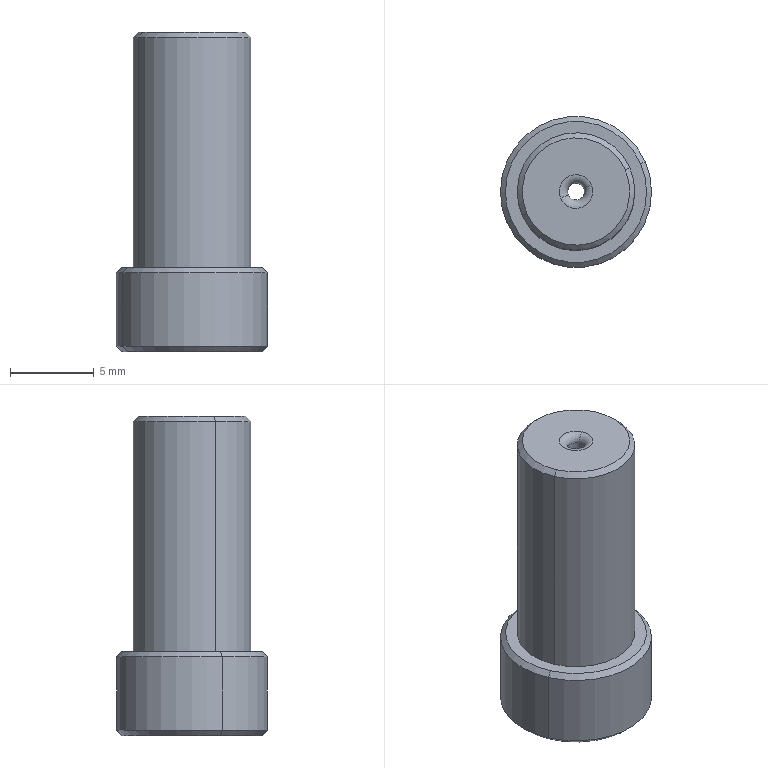Component | SolidWorks | AS-011-JG0135-1 | 1 solid | 19 faces | box 9 x 9 x 19 mm | volume 824 mm3 | cylinder 6 | cone 6 | torus 4 | plane 3 | commonest cylinder face diameters 1 x2 7 x2 9 x2
build123d program:
from build123d import *


with BuildPart() as part:
    # Sketch1 → Revolve1 (revolve)
    with BuildSketch(Plane.XY, mode=Mode.PRIVATE) as revolve1_sk:
        with BuildLine():
            Line((-4.938, 0.5), (-20.438, 0.5))
            ThreePointArc((-20.438, 0.5), (-20.792, 0.6464), (-20.938, 1))
            Line((-20.938, 1), (-20.938, 3.2))
            Line((-20.938, 3.2), (-20.638, 3.5))
            Line((-20.638, 3.5), (-6.938, 3.5))
            Line((-6.938, 3.5), (-6.938, 4.2))
            Line((-6.938, 4.2), (-6.638, 4.5))
            Line((-6.638, 4.5), (-2.238, 4.5))
            Line((-2.238, 4.5), (-1.938, 4.2))
            Line((-1.938, 4.2), (-1.938, 3.5))
            ThreePointArc((-1.938, 3.5), (-2.817, 1.379), (-4.938, 0.5))
        make_face()
    revolve(revolve1_sk.sketch.rotate(Axis((-20.938, 0, 0), (1, 0, 0)), 90), axis=Axis((-20.938, 0, 0), (1, 0, 0)))


solid = part.part

# Placed as in the assembly
solid = solid.moved(Location((-15, -28, -44.438), (0, 90, 0)))
STEP:
#1=COLOUR_RGB('',0.7922,0.8196,0.9333);
#2=FILL_AREA_STYLE_COLOUR('',#1);
#3=FILL_AREA_STYLE('',(#2));
#4=SURFACE_STYLE_FILL_AREA(#3);
#5=SURFACE_SIDE_STYLE('',(#4));
#6=SURFACE_STYLE_USAGE(.BOTH.,#5);
#7=PRESENTATION_STYLE_ASSIGNMENT((#6));
#8=CARTESIAN_POINT('',(-0.6086,-1.11,-1.555));
#9=VERTEX_POINT('',#8);
#10=CARTESIAN_POINT('',(-0.5725,-1.094,-1.555));
#11=VERTEX_POINT('',#10);
#12=CARTESIAN_POINT('',(-0.5906,-1.102,-1.555));
#13=DIRECTION('',(0.,0.,1.));
#14=DIRECTION('',(0.9157,0.4019,0.));
#15=AXIS2_PLACEMENT_3D('',#12,#13,#14);
#16=CIRCLE('',#15,0.01969);
#17=EDGE_CURVE('',#9,#11,#16,.T.);
#18=ORIENTED_EDGE('',*,*,#17,.F.);
#19=CARTESIAN_POINT('',(-0.6086,-1.11,-0.9449));
#20=VERTEX_POINT('',#19);
#21=CARTESIAN_POINT('',(-0.6086,-1.11,-0.9252));
#22=DIRECTION('',(0.,0.,1.));
#23=VECTOR('',#22,39.37);
#24=LINE('',#21,#23);
#25=EDGE_CURVE('',#9,#20,#24,.T.);
#26=ORIENTED_EDGE('',*,*,#25,.T.);
#27=CARTESIAN_POINT('',(-0.5725,-1.094,-0.9449));
#28=VERTEX_POINT('',#27);
#29=CARTESIAN_POINT('',(-0.5906,-1.102,-0.9449));
#30=DIRECTION('',(0.,0.,1.));
#31=DIRECTION('',(0.9157,0.4019,0.));
#32=AXIS2_PLACEMENT_3D('',#29,#30,#31);
#33=CIRCLE('',#32,0.01969);
#34=EDGE_CURVE('',#20,#28,#33,.T.);
#35=ORIENTED_EDGE('',*,*,#34,.T.);
#36=CARTESIAN_POINT('',(-0.5725,-1.094,-0.9252));
#37=DIRECTION('',(0.,0.,1.));
#38=VECTOR('',#37,39.37);
#39=LINE('',#36,#38);
#40=EDGE_CURVE('',#11,#28,#39,.T.);
#41=ORIENTED_EDGE('',*,*,#40,.F.);
#42=EDGE_LOOP('',(#18,#26,#35,#41));
#43=FACE_OUTER_BOUND('',#42,.T.);
#44=CARTESIAN_POINT('',(-0.5906,-1.102,-0.9252));
#45=DIRECTION('',(0.,0.,1.));
#46=DIRECTION('',(0.9157,0.4019,0.));
#47=AXIS2_PLACEMENT_3D('',#44,#45,#46);
#48=CYLINDRICAL_SURFACE('',#47,0.01969);
#49=ADVANCED_FACE('',(#43),#48,.F.);
#50=CARTESIAN_POINT('',(-0.5545,-1.087,-0.9252));
#51=VERTEX_POINT('',#50);
#52=CARTESIAN_POINT('',(-0.6266,-1.118,-0.9252));
#53=VERTEX_POINT('',#52);
#54=CARTESIAN_POINT('',(-0.5906,-1.102,-0.9252));
#55=DIRECTION('',(0.,0.,1.));
#56=DIRECTION('',(0.9157,0.4019,0.));
#57=AXIS2_PLACEMENT_3D('',#54,#55,#56);
#58=CIRCLE('',#57,0.03937);
#59=EDGE_CURVE('',#51,#53,#58,.T.);
#60=ORIENTED_EDGE('',*,*,#59,.T.);
#61=CARTESIAN_POINT('',(-0.6266,-1.118,-0.9449));
#62=DIRECTION('',(-0.4019,0.9157,-0.));
#63=DIRECTION('',(-0.9157,-0.4019,0.));
#64=AXIS2_PLACEMENT_3D('',#61,#62,#63);
#65=CIRCLE('',#64,0.01969);
#66=EDGE_CURVE('',#53,#20,#65,.T.);
#67=ORIENTED_EDGE('',*,*,#66,.T.);
#68=CARTESIAN_POINT('',(-0.5906,-1.102,-0.9449));
#69=DIRECTION('',(0.,0.,1.));
#70=DIRECTION('',(0.9157,0.4019,0.));
#71=AXIS2_PLACEMENT_3D('',#68,#69,#70);
#72=CIRCLE('',#71,0.01969);
#73=EDGE_CURVE('',#28,#20,#72,.T.);
#74=ORIENTED_EDGE('',*,*,#73,.F.);
#75=CARTESIAN_POINT('',(-0.5545,-1.087,-0.9449));
#76=DIRECTION('',(0.4019,-0.9157,0.));
#77=DIRECTION('',(0.9157,0.4019,0.));
#78=AXIS2_PLACEMENT_3D('',#75,#76,#77);
#79=CIRCLE('',#78,0.01969);
#80=EDGE_CURVE('',#51,#28,#79,.T.);
#81=ORIENTED_EDGE('',*,*,#80,.F.);
#82=EDGE_LOOP('',(#60,#67,#74,#81));
#83=FACE_OUTER_BOUND('',#82,.T.);
#84=CARTESIAN_POINT('',(-0.5906,-1.102,-0.9449));
#85=DIRECTION('',(0.,0.,1.));
#86=DIRECTION('',(0.9157,0.4019,-0.));
#87=AXIS2_PLACEMENT_3D('',#84,#85,#86);
#88=TOROIDAL_SURFACE('',#87,0.03937,0.01969);
#89=ADVANCED_FACE('',(#83),#88,.T.);
#90=CARTESIAN_POINT('',(-0.4752,-1.052,-0.9252));
#91=VERTEX_POINT('',#90);
#92=CARTESIAN_POINT('',(-0.7059,-1.153,-0.9252));
#93=VERTEX_POINT('',#92);
#94=CARTESIAN_POINT('',(-0.5906,-1.102,-0.9252));
#95=DIRECTION('',(0.,0.,1.));
#96=DIRECTION('',(0.9157,0.4019,0.));
#97=AXIS2_PLACEMENT_3D('',#94,#95,#96);
#98=CIRCLE('',#97,0.126);
#99=EDGE_CURVE('',#91,#93,#98,.T.);
#100=ORIENTED_EDGE('',*,*,#99,.F.);
#101=CARTESIAN_POINT('',(-0.4644,-1.047,-0.937));
#102=VERTEX_POINT('',#101);
#103=CARTESIAN_POINT('',(-0.4644,-1.047,-0.937));
#104=DIRECTION('',(0.6475,0.2842,-0.7071));
#105=VECTOR('',#104,39.37);
#106=LINE('',#103,#105);
#107=EDGE_CURVE('',#91,#102,#106,.T.);
#108=ORIENTED_EDGE('',*,*,#107,.T.);
#109=CARTESIAN_POINT('',(-0.7167,-1.158,-0.937));
#110=VERTEX_POINT('',#109);
#111=CARTESIAN_POINT('',(-0.5906,-1.102,-0.937));
#112=DIRECTION('',(0.,0.,1.));
#113=DIRECTION('',(0.9157,0.4019,0.));
#114=AXIS2_PLACEMENT_3D('',#111,#112,#113);
#115=CIRCLE('',#114,0.1378);
#116=EDGE_CURVE('',#102,#110,#115,.T.);
#117=ORIENTED_EDGE('',*,*,#116,.T.);
#118=CARTESIAN_POINT('',(-0.7167,-1.158,-0.937));
#119=DIRECTION('',(-0.6475,-0.2842,-0.7071));
#120=VECTOR('',#119,39.37);
#121=LINE('',#118,#120);
#122=EDGE_CURVE('',#93,#110,#121,.T.);
#123=ORIENTED_EDGE('',*,*,#122,.F.);
#124=EDGE_LOOP('',(#100,#108,#117,#123));
#125=FACE_OUTER_BOUND('',#124,.T.);
#126=CARTESIAN_POINT('',(-0.5906,-1.102,-0.937));
#127=DIRECTION('',(-0.,-0.,-1.));
#128=DIRECTION('',(-0.9157,-0.4019,0.));
#129=AXIS2_PLACEMENT_3D('',#126,#127,#128);
#130=CONICAL_SURFACE('',#129,0.1378,0.7854);
#131=ADVANCED_FACE('',(#125),#130,.T.);
#132=CARTESIAN_POINT('',(-0.4644,-1.047,-1.476));
#133=VERTEX_POINT('',#132);
#134=CARTESIAN_POINT('',(-0.7167,-1.158,-1.476));
#135=VERTEX_POINT('',#134);
#136=CARTESIAN_POINT('',(-0.5906,-1.102,-1.476));
#137=DIRECTION('',(0.,0.,1.));
#138=DIRECTION('',(0.9157,0.4019,0.));
#139=AXIS2_PLACEMENT_3D('',#136,#137,#138);
#140=CIRCLE('',#139,0.1378);
#141=EDGE_CURVE('',#133,#135,#140,.T.);
#142=ORIENTED_EDGE('',*,*,#141,.T.);
#143=CARTESIAN_POINT('',(-0.7167,-1.158,-0.9252));
#144=DIRECTION('',(0.,0.,1.));
#145=VECTOR('',#144,39.37);
#146=LINE('',#143,#145);
#147=EDGE_CURVE('',#135,#110,#146,.T.);
#148=ORIENTED_EDGE('',*,*,#147,.T.);
#149=ORIENTED_EDGE('',*,*,#116,.F.);
#150=CARTESIAN_POINT('',(-0.4644,-1.047,-0.9252));
#151=DIRECTION('',(0.,0.,1.));
#152=VECTOR('',#151,39.37);
#153=LINE('',#150,#152);
#154=EDGE_CURVE('',#133,#102,#153,.T.);
#155=ORIENTED_EDGE('',*,*,#154,.F.);
#156=EDGE_LOOP('',(#142,#148,#149,#155));
#157=FACE_OUTER_BOUND('',#156,.T.);
#158=CARTESIAN_POINT('',(-0.5906,-1.102,-0.9252));
#159=DIRECTION('',(0.,0.,1.));
#160=DIRECTION('',(0.9157,0.4019,0.));
#161=AXIS2_PLACEMENT_3D('',#158,#159,#160);
#162=CYLINDRICAL_SURFACE('',#161,0.1378);
#163=ADVANCED_FACE('',(#157),#162,.T.);
#164=CARTESIAN_POINT('',(-0.4391,-1.036,-1.476));
#165=VERTEX_POINT('',#164);
#166=CARTESIAN_POINT('',(-0.742,-1.169,-1.476));
#167=VERTEX_POINT('',#166);
#168=CARTESIAN_POINT('',(-0.5906,-1.102,-1.476));
#169=DIRECTION('',(0.,0.,1.));
#170=DIRECTION('',(0.9157,0.4019,0.));
#171=AXIS2_PLACEMENT_3D('',#168,#169,#170);
#172=CIRCLE('',#171,0.1654);
#173=EDGE_CURVE('',#165,#167,#172,.T.);
#174=ORIENTED_EDGE('',*,*,#173,.F.);
#175=CARTESIAN_POINT('',(-0.4283,-1.031,-1.488));
#176=VERTEX_POINT('',#175);
#177=CARTESIAN_POINT('',(-0.4283,-1.031,-1.488));
#178=DIRECTION('',(0.6475,0.2842,-0.7071));
#179=VECTOR('',#178,39.37);
#180=LINE('',#177,#179);
#181=EDGE_CURVE('',#165,#176,#180,.T.);
#182=ORIENTED_EDGE('',*,*,#181,.T.);
#183=CARTESIAN_POINT('',(-0.7528,-1.174,-1.488));
#184=VERTEX_POINT('',#183);
#185=CARTESIAN_POINT('',(-0.5906,-1.102,-1.488));
#186=DIRECTION('',(0.,0.,1.));
#187=DIRECTION('',(0.9157,0.4019,0.));
#188=AXIS2_PLACEMENT_3D('',#185,#186,#187);
#189=CIRCLE('',#188,0.1772);
#190=EDGE_CURVE('',#176,#184,#189,.T.);
#191=ORIENTED_EDGE('',*,*,#190,.T.);
#192=CARTESIAN_POINT('',(-0.7528,-1.174,-1.488));
#193=DIRECTION('',(-0.6475,-0.2842,-0.7071));
#194=VECTOR('',#193,39.37);
#195=LINE('',#192,#194);
#196=EDGE_CURVE('',#167,#184,#195,.T.);
#197=ORIENTED_EDGE('',*,*,#196,.F.);
#198=EDGE_LOOP('',(#174,#182,#191,#197));
#199=FACE_OUTER_BOUND('',#198,.T.);
#200=CARTESIAN_POINT('',(-0.5906,-1.102,-1.488));
#201=DIRECTION('',(-0.,-0.,-1.));
#202=DIRECTION('',(-0.9157,-0.4019,0.));
#203=AXIS2_PLACEMENT_3D('',#200,#201,#202);
#204=CONICAL_SURFACE('',#203,0.1772,0.7854);
#205=ADVANCED_FACE('',(#199),#204,.T.);
#206=CARTESIAN_POINT('',(-0.4283,-1.031,-1.661));
#207=VERTEX_POINT('',#206);
#208=CARTESIAN_POINT('',(-0.7528,-1.174,-1.661));
#209=VERTEX_POINT('',#208);
#210=CARTESIAN_POINT('',(-0.5906,-1.102,-1.661));
#211=DIRECTION('',(0.,0.,1.));
#212=DIRECTION('',(0.9157,0.4019,0.));
#213=AXIS2_PLACEMENT_3D('',#210,#211,#212);
#214=CIRCLE('',#213,0.1772);
#215=EDGE_CURVE('',#207,#209,#214,.T.);
#216=ORIENTED_EDGE('',*,*,#215,.T.);
#217=CARTESIAN_POINT('',(-0.7528,-1.174,-0.9252));
#218=DIRECTION('',(0.,0.,1.));
#219=VECTOR('',#218,39.37);
#220=LINE('',#217,#219);
#221=EDGE_CURVE('',#209,#184,#220,.T.);
#222=ORIENTED_EDGE('',*,*,#221,.T.);
#223=ORIENTED_EDGE('',*,*,#190,.F.);
#224=CARTESIAN_POINT('',(-0.4283,-1.031,-0.9252));
#225=DIRECTION('',(0.,0.,1.));
#226=VECTOR('',#225,39.37);
#227=LINE('',#224,#226);
#228=EDGE_CURVE('',#207,#176,#227,.T.);
#229=ORIENTED_EDGE('',*,*,#228,.F.);
#230=EDGE_LOOP('',(#216,#222,#223,#229));
#231=FACE_OUTER_BOUND('',#230,.T.);
#232=CARTESIAN_POINT('',(-0.5906,-1.102,-0.9252));
#233=DIRECTION('',(0.,0.,1.));
#234=DIRECTION('',(0.9157,0.4019,0.));
#235=AXIS2_PLACEMENT_3D('',#232,#233,#234);
#236=CYLINDRICAL_SURFACE('',#235,0.1772);
#237=ADVANCED_FACE('',(#231),#236,.T.);
#238=CARTESIAN_POINT('',(-0.4391,-1.036,-1.673));
#239=VERTEX_POINT('',#238);
#240=CARTESIAN_POINT('',(-0.742,-1.169,-1.673));
#241=VERTEX_POINT('',#240);
#242=CARTESIAN_POINT('',(-0.5906,-1.102,-1.673));
#243=DIRECTION('',(0.,0.,1.));
#244=DIRECTION('',(0.9157,0.4019,0.));
#245=AXIS2_PLACEMENT_3D('',#242,#243,#244);
#246=CIRCLE('',#245,0.1654);
#247=EDGE_CURVE('',#239,#241,#246,.T.);
#248=ORIENTED_EDGE('',*,*,#247,.T.);
#249=CARTESIAN_POINT('',(-0.742,-1.169,-1.673));
#250=DIRECTION('',(-0.6475,-0.2842,0.7071));
#251=VECTOR('',#250,39.37);
#252=LINE('',#249,#251);
#253=EDGE_CURVE('',#241,#209,#252,.T.);
#254=ORIENTED_EDGE('',*,*,#253,.T.);
#255=ORIENTED_EDGE('',*,*,#215,.F.);
#256=CARTESIAN_POINT('',(-0.4391,-1.036,-1.673));
#257=DIRECTION('',(0.6475,0.2842,0.7071));
#258=VECTOR('',#257,39.37);
#259=LINE('',#256,#258);
#260=EDGE_CURVE('',#239,#207,#259,.T.);
#261=ORIENTED_EDGE('',*,*,#260,.F.);
#262=EDGE_LOOP('',(#248,#254,#255,#261));
#263=FACE_OUTER_BOUND('',#262,.T.);
#264=CARTESIAN_POINT('',(-0.5906,-1.102,-1.673));
#265=DIRECTION('',(0.,0.,1.));
#266=DIRECTION('',(0.9157,0.4019,0.));
#267=AXIS2_PLACEMENT_3D('',#264,#265,#266);
#268=CONICAL_SURFACE('',#267,0.1654,0.7854);
#269=ADVANCED_FACE('',(#263),#268,.T.);
#270=CARTESIAN_POINT('',(-0.5906,-1.102,-1.555));
#271=DIRECTION('',(0.,0.,1.));
#272=DIRECTION('',(0.9157,0.4019,0.));
#273=AXIS2_PLACEMENT_3D('',#270,#271,#272);
#274=CIRCLE('',#273,0.01969);
#275=EDGE_CURVE('',#11,#9,#274,.T.);
#276=ORIENTED_EDGE('',*,*,#275,.T.);
#277=CARTESIAN_POINT('',(-0.7167,-1.158,-1.673));
#278=VERTEX_POINT('',#277);
#279=CARTESIAN_POINT('',(-0.7167,-1.158,-1.555));
#280=DIRECTION('',(-0.4019,0.9157,-0.));
#281=DIRECTION('',(-0.9157,-0.4019,0.));
#282=AXIS2_PLACEMENT_3D('',#279,#280,#281);
#283=CIRCLE('',#282,0.1181);
#284=EDGE_CURVE('',#9,#278,#283,.T.);
#285=ORIENTED_EDGE('',*,*,#284,.T.);
#286=CARTESIAN_POINT('',(-0.4644,-1.047,-1.673));
#287=VERTEX_POINT('',#286);
#288=CARTESIAN_POINT('',(-0.5906,-1.102,-1.673));
#289=DIRECTION('',(0.,0.,1.));
#290=DIRECTION('',(0.9157,0.4019,0.));
#291=AXIS2_PLACEMENT_3D('',#288,#289,#290);
#292=CIRCLE('',#291,0.1378);
#293=EDGE_CURVE('',#287,#278,#292,.T.);
#294=ORIENTED_EDGE('',*,*,#293,.F.);
#295=CARTESIAN_POINT('',(-0.4644,-1.047,-1.555));
#296=DIRECTION('',(0.4019,-0.9157,0.));
#297=DIRECTION('',(0.9157,0.4019,0.));
#298=AXIS2_PLACEMENT_3D('',#295,#296,#297);
#299=CIRCLE('',#298,0.1181);
#300=EDGE_CURVE('',#11,#287,#299,.T.);
#301=ORIENTED_EDGE('',*,*,#300,.F.);
#302=EDGE_LOOP('',(#276,#285,#294,#301));
#303=FACE_OUTER_BOUND('',#302,.T.);
#304=CARTESIAN_POINT('',(-0.5906,-1.102,-1.555));
#305=DIRECTION('',(0.,0.,1.));
#306=DIRECTION('',(0.9157,0.4019,-0.));
#307=AXIS2_PLACEMENT_3D('',#304,#305,#306);
#308=TOROIDAL_SURFACE('',#307,0.1378,0.1181);
#309=ADVANCED_FACE('',(#303),#308,.T.);
#310=ORIENTED_EDGE('',*,*,#284,.F.);
#311=ORIENTED_EDGE('',*,*,#17,.T.);
#312=ORIENTED_EDGE('',*,*,#300,.T.);
#313=CARTESIAN_POINT('',(-0.5906,-1.102,-1.673));
#314=DIRECTION('',(0.,0.,1.));
#315=DIRECTION('',(0.9157,0.4019,0.));
#316=AXIS2_PLACEMENT_3D('',#313,#314,#315);
#317=CIRCLE('',#316,0.1378);
#318=EDGE_CURVE('',#278,#287,#317,.T.);
#319=ORIENTED_EDGE('',*,*,#318,.F.);
#320=EDGE_LOOP('',(#310,#311,#312,#319));
#321=FACE_OUTER_BOUND('',#320,.T.);
#322=CARTESIAN_POINT('',(-0.5906,-1.102,-1.555));
#323=DIRECTION('',(0.,0.,1.));
#324=DIRECTION('',(0.9157,0.4019,-0.));
#325=AXIS2_PLACEMENT_3D('',#322,#323,#324);
#326=TOROIDAL_SURFACE('',#325,0.1378,0.1181);
#327=ADVANCED_FACE('',(#321),#326,.T.);
#328=ORIENTED_EDGE('',*,*,#247,.F.);
#329=CARTESIAN_POINT('',(-0.5906,-1.102,-1.673));
#330=DIRECTION('',(0.,0.,1.));
#331=DIRECTION('',(0.9157,0.4019,0.));
#332=AXIS2_PLACEMENT_3D('',#329,#330,#331);
#333=CIRCLE('',#332,0.1654);
#334=EDGE_CURVE('',#241,#239,#333,.T.);
#335=ORIENTED_EDGE('',*,*,#334,.F.);
#336=EDGE_LOOP('',(#328,#335));
#337=FACE_OUTER_BOUND('',#336,.T.);
#338=ORIENTED_EDGE('',*,*,#293,.T.);
#339=ORIENTED_EDGE('',*,*,#318,.T.);
#340=EDGE_LOOP('',(#338,#339));
#341=FACE_BOUND('',#340,.T.);
#342=CARTESIAN_POINT('',(-0.657,-0.951,-1.673));
#343=DIRECTION('',(-0.,0.,1.));
#344=DIRECTION('',(0.9157,0.4019,-0.));
#345=AXIS2_PLACEMENT_3D('',#342,#343,#344);
#346=PLANE('',#345);
#347=ADVANCED_FACE('',(#337,#341),#346,.F.);
#348=ORIENTED_EDGE('',*,*,#253,.F.);
#349=ORIENTED_EDGE('',*,*,#334,.T.);
#350=ORIENTED_EDGE('',*,*,#260,.T.);
#351=CARTESIAN_POINT('',(-0.5906,-1.102,-1.661));
#352=DIRECTION('',(0.,0.,1.));
#353=DIRECTION('',(0.9157,0.4019,0.));
#354=AXIS2_PLACEMENT_3D('',#351,#352,#353);
#355=CIRCLE('',#354,0.1772);
#356=EDGE_CURVE('',#209,#207,#355,.T.);
#357=ORIENTED_EDGE('',*,*,#356,.F.);
#358=EDGE_LOOP('',(#348,#349,#350,#357));
#359=FACE_OUTER_BOUND('',#358,.T.);
#360=CARTESIAN_POINT('',(-0.5906,-1.102,-1.673));
#361=DIRECTION('',(0.,0.,1.));
#362=DIRECTION('',(0.9157,0.4019,0.));
#363=AXIS2_PLACEMENT_3D('',#360,#361,#362);
#364=CONICAL_SURFACE('',#363,0.1654,0.7854);
#365=ADVANCED_FACE('',(#359),#364,.T.);
#366=ORIENTED_EDGE('',*,*,#221,.F.);
#367=ORIENTED_EDGE('',*,*,#356,.T.);
#368=ORIENTED_EDGE('',*,*,#228,.T.);
#369=CARTESIAN_POINT('',(-0.5906,-1.102,-1.488));
#370=DIRECTION('',(0.,0.,1.));
#371=DIRECTION('',(0.9157,0.4019,0.));
#372=AXIS2_PLACEMENT_3D('',#369,#370,#371);
#373=CIRCLE('',#372,0.1772);
#374=EDGE_CURVE('',#184,#176,#373,.T.);
#375=ORIENTED_EDGE('',*,*,#374,.F.);
#376=EDGE_LOOP('',(#366,#367,#368,#375));
#377=FACE_OUTER_BOUND('',#376,.T.);
#378=CARTESIAN_POINT('',(-0.5906,-1.102,-0.9252));
#379=DIRECTION('',(0.,0.,1.));
#380=DIRECTION('',(0.9157,0.4019,0.));
#381=AXIS2_PLACEMENT_3D('',#378,#379,#380);
#382=CYLINDRICAL_SURFACE('',#381,0.1772);
#383=ADVANCED_FACE('',(#377),#382,.T.);
#384=ORIENTED_EDGE('',*,*,#181,.F.);
#385=CARTESIAN_POINT('',(-0.5906,-1.102,-1.476));
#386=DIRECTION('',(0.,0.,1.));
#387=DIRECTION('',(0.9157,0.4019,0.));
#388=AXIS2_PLACEMENT_3D('',#385,#386,#387);
#389=CIRCLE('',#388,0.1654);
#390=EDGE_CURVE('',#167,#165,#389,.T.);
#391=ORIENTED_EDGE('',*,*,#390,.F.);
#392=ORIENTED_EDGE('',*,*,#196,.T.);
#393=ORIENTED_EDGE('',*,*,#374,.T.);
#394=EDGE_LOOP('',(#384,#391,#392,#393));
#395=FACE_OUTER_BOUND('',#394,.T.);
#396=CARTESIAN_POINT('',(-0.5906,-1.102,-1.488));
#397=DIRECTION('',(-0.,-0.,-1.));
#398=DIRECTION('',(-0.9157,-0.4019,0.));
#399=AXIS2_PLACEMENT_3D('',#396,#397,#398);
#400=CONICAL_SURFACE('',#399,0.1772,0.7854);
#401=ADVANCED_FACE('',(#395),#400,.T.);
#402=ORIENTED_EDGE('',*,*,#141,.F.);
#403=CARTESIAN_POINT('',(-0.5906,-1.102,-1.476));
#404=DIRECTION('',(0.,0.,1.));
#405=DIRECTION('',(0.9157,0.4019,0.));
#406=AXIS2_PLACEMENT_3D('',#403,#404,#405);
#407=CIRCLE('',#406,0.1378);
#408=EDGE_CURVE('',#135,#133,#407,.T.);
#409=ORIENTED_EDGE('',*,*,#408,.F.);
#410=EDGE_LOOP('',(#402,#409));
#411=FACE_BOUND('',#410,.T.);
#412=ORIENTED_EDGE('',*,*,#390,.T.);
#413=ORIENTED_EDGE('',*,*,#173,.T.);
#414=EDGE_LOOP('',(#412,#413));
#415=FACE_OUTER_BOUND('',#414,.T.);
#416=CARTESIAN_POINT('',(-0.6459,-0.9762,-1.476));
#417=DIRECTION('',(0.,-0.,-1.));
#418=DIRECTION('',(-0.9157,-0.4019,0.));
#419=AXIS2_PLACEMENT_3D('',#416,#417,#418);
#420=PLANE('',#419);
#421=ADVANCED_FACE('',(#411,#415),#420,.F.);
#422=ORIENTED_EDGE('',*,*,#147,.F.);
#423=ORIENTED_EDGE('',*,*,#408,.T.);
#424=ORIENTED_EDGE('',*,*,#154,.T.);
#425=CARTESIAN_POINT('',(-0.5906,-1.102,-0.937));
#426=DIRECTION('',(0.,0.,1.));
#427=DIRECTION('',(0.9157,0.4019,0.));
#428=AXIS2_PLACEMENT_3D('',#425,#426,#427);
#429=CIRCLE('',#428,0.1378);
#430=EDGE_CURVE('',#110,#102,#429,.T.);
#431=ORIENTED_EDGE('',*,*,#430,.F.);
#432=EDGE_LOOP('',(#422,#423,#424,#431));
#433=FACE_OUTER_BOUND('',#432,.T.);
#434=CARTESIAN_POINT('',(-0.5906,-1.102,-0.9252));
#435=DIRECTION('',(0.,0.,1.));
#436=DIRECTION('',(0.9157,0.4019,0.));
#437=AXIS2_PLACEMENT_3D('',#434,#435,#436);
#438=CYLINDRICAL_SURFACE('',#437,0.1378);
#439=ADVANCED_FACE('',(#433),#438,.T.);
#440=ORIENTED_EDGE('',*,*,#107,.F.);
#441=CARTESIAN_POINT('',(-0.5906,-1.102,-0.9252));
#442=DIRECTION('',(0.,0.,1.));
#443=DIRECTION('',(0.9157,0.4019,0.));
#444=AXIS2_PLACEMENT_3D('',#441,#442,#443);
#445=CIRCLE('',#444,0.126);
#446=EDGE_CURVE('',#93,#91,#445,.T.);
#447=ORIENTED_EDGE('',*,*,#446,.F.);
#448=ORIENTED_EDGE('',*,*,#122,.T.);
#449=ORIENTED_EDGE('',*,*,#430,.T.);
#450=EDGE_LOOP('',(#440,#447,#448,#449));
#451=FACE_OUTER_BOUND('',#450,.T.);
#452=CARTESIAN_POINT('',(-0.5906,-1.102,-0.937));
#453=DIRECTION('',(-0.,-0.,-1.));
#454=DIRECTION('',(-0.9157,-0.4019,0.));
#455=AXIS2_PLACEMENT_3D('',#452,#453,#454);
#456=CONICAL_SURFACE('',#455,0.1378,0.7854);
#457=ADVANCED_FACE('',(#451),#456,.T.);
#458=ORIENTED_EDGE('',*,*,#59,.F.);
#459=CARTESIAN_POINT('',(-0.5906,-1.102,-0.9252));
#460=DIRECTION('',(0.,0.,1.));
#461=DIRECTION('',(0.9157,0.4019,0.));
#462=AXIS2_PLACEMENT_3D('',#459,#460,#461);
#463=CIRCLE('',#462,0.03937);
#464=EDGE_CURVE('',#53,#51,#463,.T.);
#465=ORIENTED_EDGE('',*,*,#464,.F.);
#466=EDGE_LOOP('',(#458,#465));
#467=FACE_BOUND('',#466,.T.);
#468=ORIENTED_EDGE('',*,*,#446,.T.);
#469=ORIENTED_EDGE('',*,*,#99,.T.);
#470=EDGE_LOOP('',(#468,#469));
#471=FACE_OUTER_BOUND('',#470,.T.);
#472=CARTESIAN_POINT('',(-0.6412,-0.987,-0.9252));
#473=DIRECTION('',(0.,-0.,-1.));
#474=DIRECTION('',(-0.9157,-0.4019,0.));
#475=AXIS2_PLACEMENT_3D('',#472,#473,#474);
#476=PLANE('',#475);
#477=ADVANCED_FACE('',(#467,#471),#476,.F.);
#478=ORIENTED_EDGE('',*,*,#66,.F.);
#479=ORIENTED_EDGE('',*,*,#464,.T.);
#480=ORIENTED_EDGE('',*,*,#80,.T.);
#481=ORIENTED_EDGE('',*,*,#34,.F.);
#482=EDGE_LOOP('',(#478,#479,#480,#481));
#483=FACE_OUTER_BOUND('',#482,.T.);
#484=CARTESIAN_POINT('',(-0.5906,-1.102,-0.9449));
#485=DIRECTION('',(0.,0.,1.));
#486=DIRECTION('',(0.9157,0.4019,-0.));
#487=AXIS2_PLACEMENT_3D('',#484,#485,#486);
#488=TOROIDAL_SURFACE('',#487,0.03937,0.01969);
#489=ADVANCED_FACE('',(#483),#488,.T.);
#490=ORIENTED_EDGE('',*,*,#25,.F.);
#491=ORIENTED_EDGE('',*,*,#275,.F.);
#492=ORIENTED_EDGE('',*,*,#40,.T.);
#493=ORIENTED_EDGE('',*,*,#73,.T.);
#494=EDGE_LOOP('',(#490,#491,#492,#493));
#495=FACE_OUTER_BOUND('',#494,.T.);
#496=CARTESIAN_POINT('',(-0.5906,-1.102,-0.9252));
#497=DIRECTION('',(0.,0.,1.));
#498=DIRECTION('',(0.9157,0.4019,0.));
#499=AXIS2_PLACEMENT_3D('',#496,#497,#498);
#500=CYLINDRICAL_SURFACE('',#499,0.01969);
#501=ADVANCED_FACE('',(#495),#500,.F.);
#502=CLOSED_SHELL('',(#49,#89,#131,#163,#205,#237,#269,#309,#327,#347,#365,#383,#401,#421,#439,#457,#477,#489,#501));
#503=MANIFOLD_SOLID_BREP('',#502);
#504=STYLED_ITEM('',(#7),#503);
#505=PRESENTATION_LAYER_ASSIGNMENT('','',(#504));
#506=(LENGTH_UNIT()NAMED_UNIT(*)SI_UNIT($,.METRE.));
#507=LENGTH_MEASURE_WITH_UNIT(LENGTH_MEASURE(0.0254),#506);
#508=DIMENSIONAL_EXPONENTS(1.,0.,0.,0.,0.,0.,0.);
#509=(CONVERSION_BASED_UNIT('',#507)LENGTH_UNIT()NAMED_UNIT(#508));
#510=UNCERTAINTY_MEASURE_WITH_UNIT(LENGTH_MEASURE(0.00001),#509,'','');
#511=(NAMED_UNIT(*)PLANE_ANGLE_UNIT()SI_UNIT($,.RADIAN.));
#512=(NAMED_UNIT(*)SI_UNIT($,.STERADIAN.)SOLID_ANGLE_UNIT());
#513=(GEOMETRIC_REPRESENTATION_CONTEXT(3)GLOBAL_UNCERTAINTY_ASSIGNED_CONTEXT((#510))GLOBAL_UNIT_ASSIGNED_CONTEXT((#509,#511,#512))REPRESENTATION_CONTEXT('',''));
#514=MECHANICAL_DESIGN_GEOMETRIC_PRESENTATION_REPRESENTATION('',(#504),#513);
#515=CARTESIAN_POINT('',(0.,0.,0.));
#516=DIRECTION('',(0.,0.,1.));
#517=DIRECTION('',(1.,0.,0.));
#518=AXIS2_PLACEMENT_3D('',#515,#516,#517);
#519=(LENGTH_UNIT()NAMED_UNIT(*)SI_UNIT($,.METRE.));
#520=LENGTH_MEASURE_WITH_UNIT(LENGTH_MEASURE(0.0254),#519);
#521=DIMENSIONAL_EXPONENTS(1.,0.,0.,0.,0.,0.,0.);
#522=(CONVERSION_BASED_UNIT('',#520)LENGTH_UNIT()NAMED_UNIT(#521));
#523=UNCERTAINTY_MEASURE_WITH_UNIT(LENGTH_MEASURE(0.00001),#522,'','');
#524=(NAMED_UNIT(*)PLANE_ANGLE_UNIT()SI_UNIT($,.RADIAN.));
#525=(NAMED_UNIT(*)SI_UNIT($,.STERADIAN.)SOLID_ANGLE_UNIT());
#526=(GEOMETRIC_REPRESENTATION_CONTEXT(3)GLOBAL_UNCERTAINTY_ASSIGNED_CONTEXT((#523))GLOBAL_UNIT_ASSIGNED_CONTEXT((#522,#524,#525))REPRESENTATION_CONTEXT('',''));
#527=ADVANCED_BREP_SHAPE_REPRESENTATION('',(#503,#518),#526);